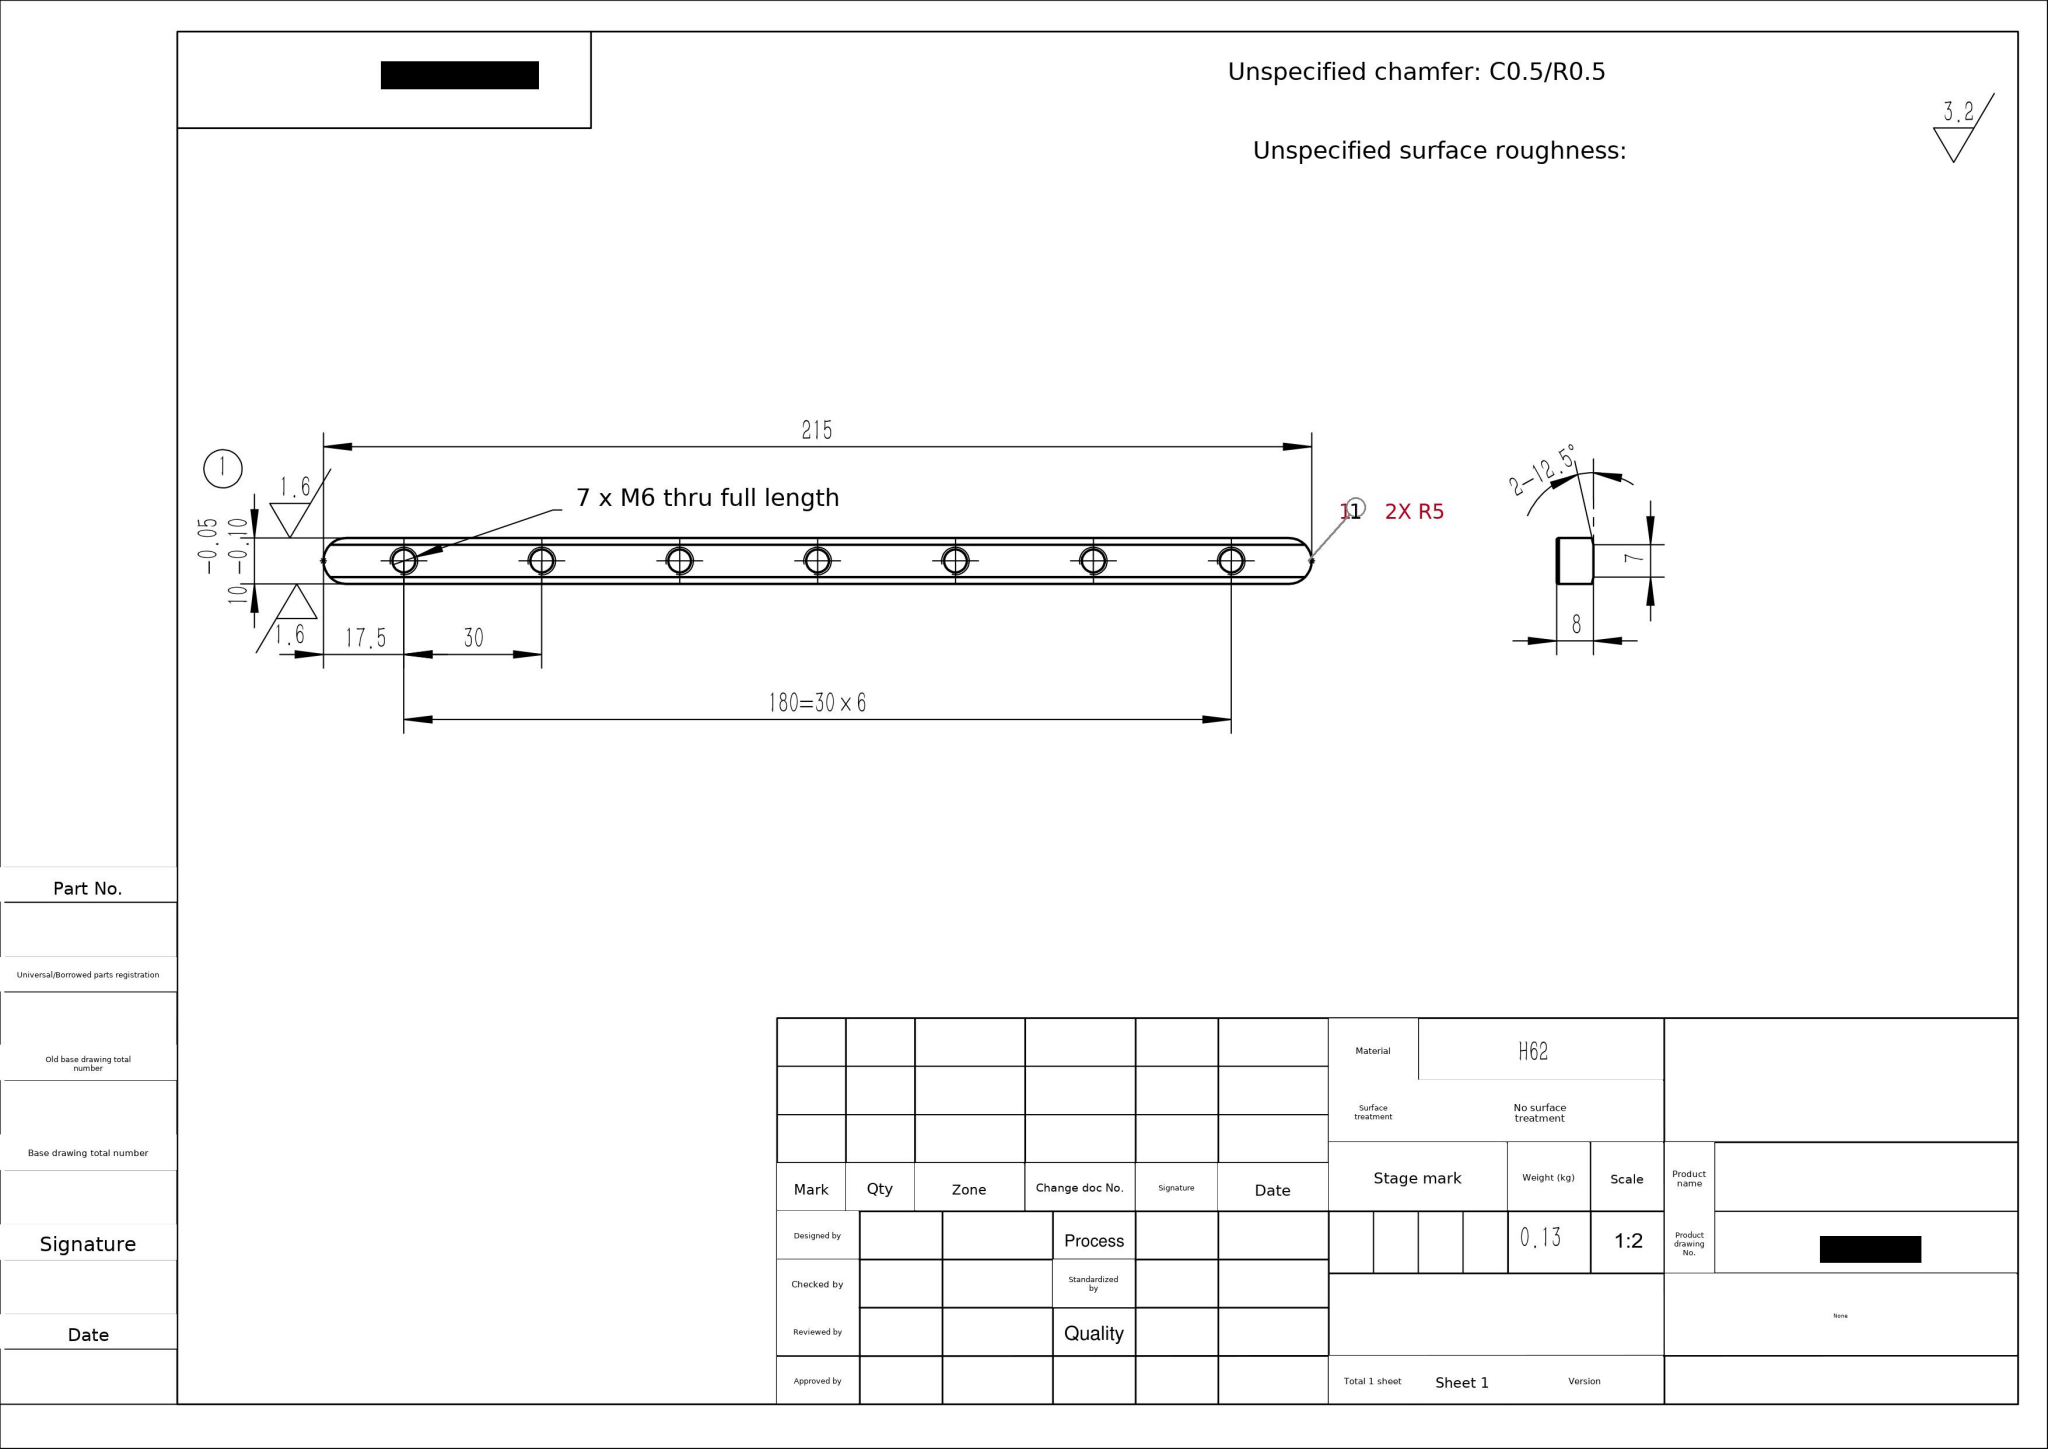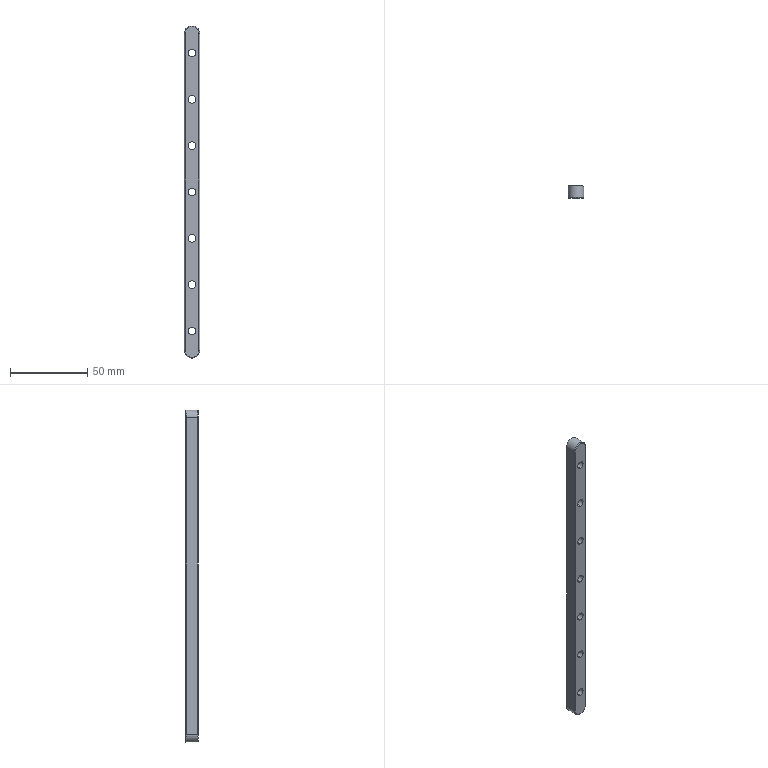Part | SolidWorks | mm | material H62 | 1 solid | 27 faces | box 10 x 8 x 215 mm | volume 15801 mm3 | cylinder 18 | plane 6 | torus 3 | commonest cylinder face diameters 5 x14 10 x2 1 x2
build123d program:
from build123d import *

# Parameters (mm, degrees)
SKETCH1_W           = 10
SKETCH1_H           = 8
BOSS_EXTRUDE1_DEPTH = 215
FILLET1_RADIUS      = 5
FILLET1_LENGTH      = 8
FILLET2_RADIUS      = 5
FILLET2_LENGTH      = 8
CUT_EXTRUDE5_DEPTH  = 216.095
FILLET3_R           = 0.5
M6_TAPPED_HOLE1_D   = 5
LPATTERN2_COUNT     = 4
LPATTERN2_PITCH     = 30
LPATTERN3_COUNT     = 4
LPATTERN3_PITCH     = 30


with BuildPart() as part:
    # Sketch1 → Boss-Extrude1 (new body)
    with BuildSketch(Plane.XY):
        Rectangle(SKETCH1_W, SKETCH1_H)
    extrude(amount=BOSS_EXTRUDE1_DEPTH)

    # Fillet1: full round fillet: the end face becomes a half cylinder, R = half its width
    fillet1_face = Plane((0, 0, 0), x_dir=(0, 1, 0), z_dir=(0, 0, -1))  # on the end face: x along it, z out of the body
    fillet1_slab = fillet1_face.offset(-FILLET1_RADIUS / 2) * Box(FILLET1_LENGTH, 2 * FILLET1_RADIUS, FILLET1_RADIUS, mode=Mode.PRIVATE)  # the body's end, R deep
    fillet1_round = Plane((0, 0, 5), x_dir=(0, 0, -1), z_dir=(0, 1, 0)) * Cylinder(FILLET1_RADIUS, FILLET1_LENGTH, mode=Mode.PRIVATE)  # its axis R under the face
    add(fillet1_slab - fillet1_round, mode=Mode.SUBTRACT)

    # Fillet2: full round fillet: the end face becomes a half cylinder, R = half its width
    fillet2_face = Plane((0, 0, 215), x_dir=(0, -1, 0), z_dir=(0, 0, 1))  # on the end face: x along it, z out of the body
    fillet2_slab = fillet2_face.offset(-FILLET2_RADIUS / 2) * Box(FILLET2_LENGTH, 2 * FILLET2_RADIUS, FILLET2_RADIUS, mode=Mode.PRIVATE)  # the body's end, R deep
    fillet2_round = Plane((0, 0, 210), x_dir=(0, 0, 1), z_dir=(0, -1, 0)) * Cylinder(FILLET2_RADIUS, FILLET2_LENGTH, mode=Mode.PRIVATE)  # its axis R under the face
    add(fillet2_slab - fillet2_round, mode=Mode.SUBTRACT)

    # Sketch6 → Cut-Extrude5 (cut, through all)
    with BuildSketch(Plane.XY):
        Polygon((-3.5, 4), (-11.769, 4), (-11.769, 2.167), align=None)
        Polygon((11.769, 4), (11.769, 2.167), (3.5, 4), align=None)
    extrude(amount=CUT_EXTRUDE5_DEPTH, mode=Mode.SUBTRACT)

    # Fillet3
    fillet3_edges = [part.edges().sort_by_distance(p)[0] for p in [
        (0, -4, 0),
        (5, -4, 107.5),
        (-5, -4, 107.5),
        (0, -4, 215),
    ]]
    fillet(fillet3_edges, radius=FILLET3_R)

    # M6 Tapped Hole1 (through all)
    with Locations(Plane(origin=(0, 4, 0), x_dir=(1, 0, 0), z_dir=(0, 1, 0))):
        with Locations((0, -107.5)):
            m6_tapped_hole1 = Hole(M6_TAPPED_HOLE1_D / 2)

    # LPattern2: M6 Tapped Hole1 ×4
    with Locations(*[(0, 0, i * LPATTERN2_PITCH) for i in range(1, LPATTERN2_COUNT)]):
        add(m6_tapped_hole1, mode=Mode.SUBTRACT)

    # LPattern3: M6 Tapped Hole1 ×4
    with Locations(*[(0, 0, -i * LPATTERN3_PITCH) for i in range(1, LPATTERN3_COUNT)]):
        add(m6_tapped_hole1, mode=Mode.SUBTRACT)


solid = part.part